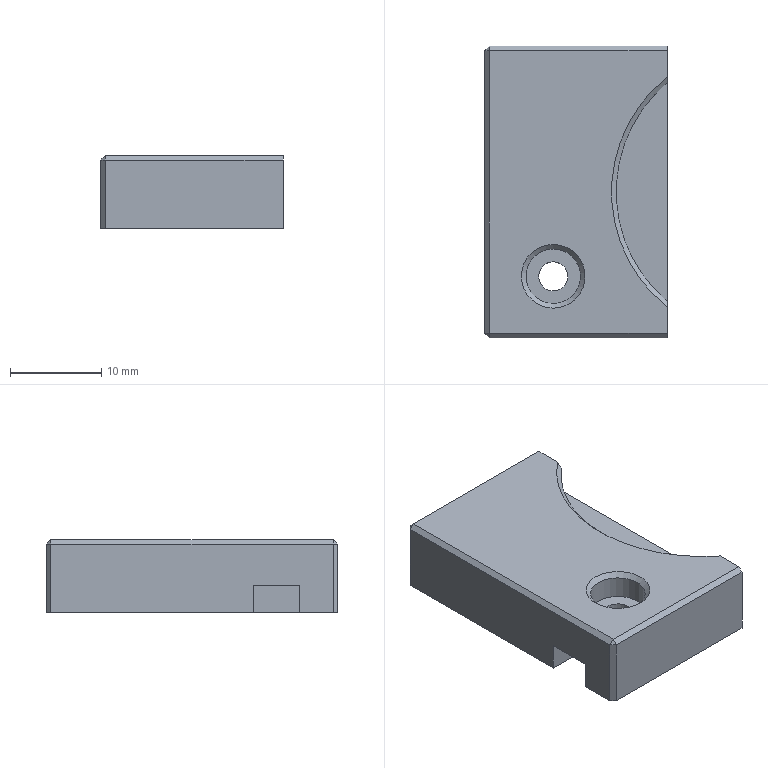Component | NX | DJZ_13_JAW | 1 solid | 55 faces | volume 3535 mm3 | plane 25 | cylinder 15 | spline 6 | sphere 5 | cone 2 | torus 2 | commonest cylinder face diameters 1 x11 3.2 x1 6 x1 31.2 x1 37.2 x1